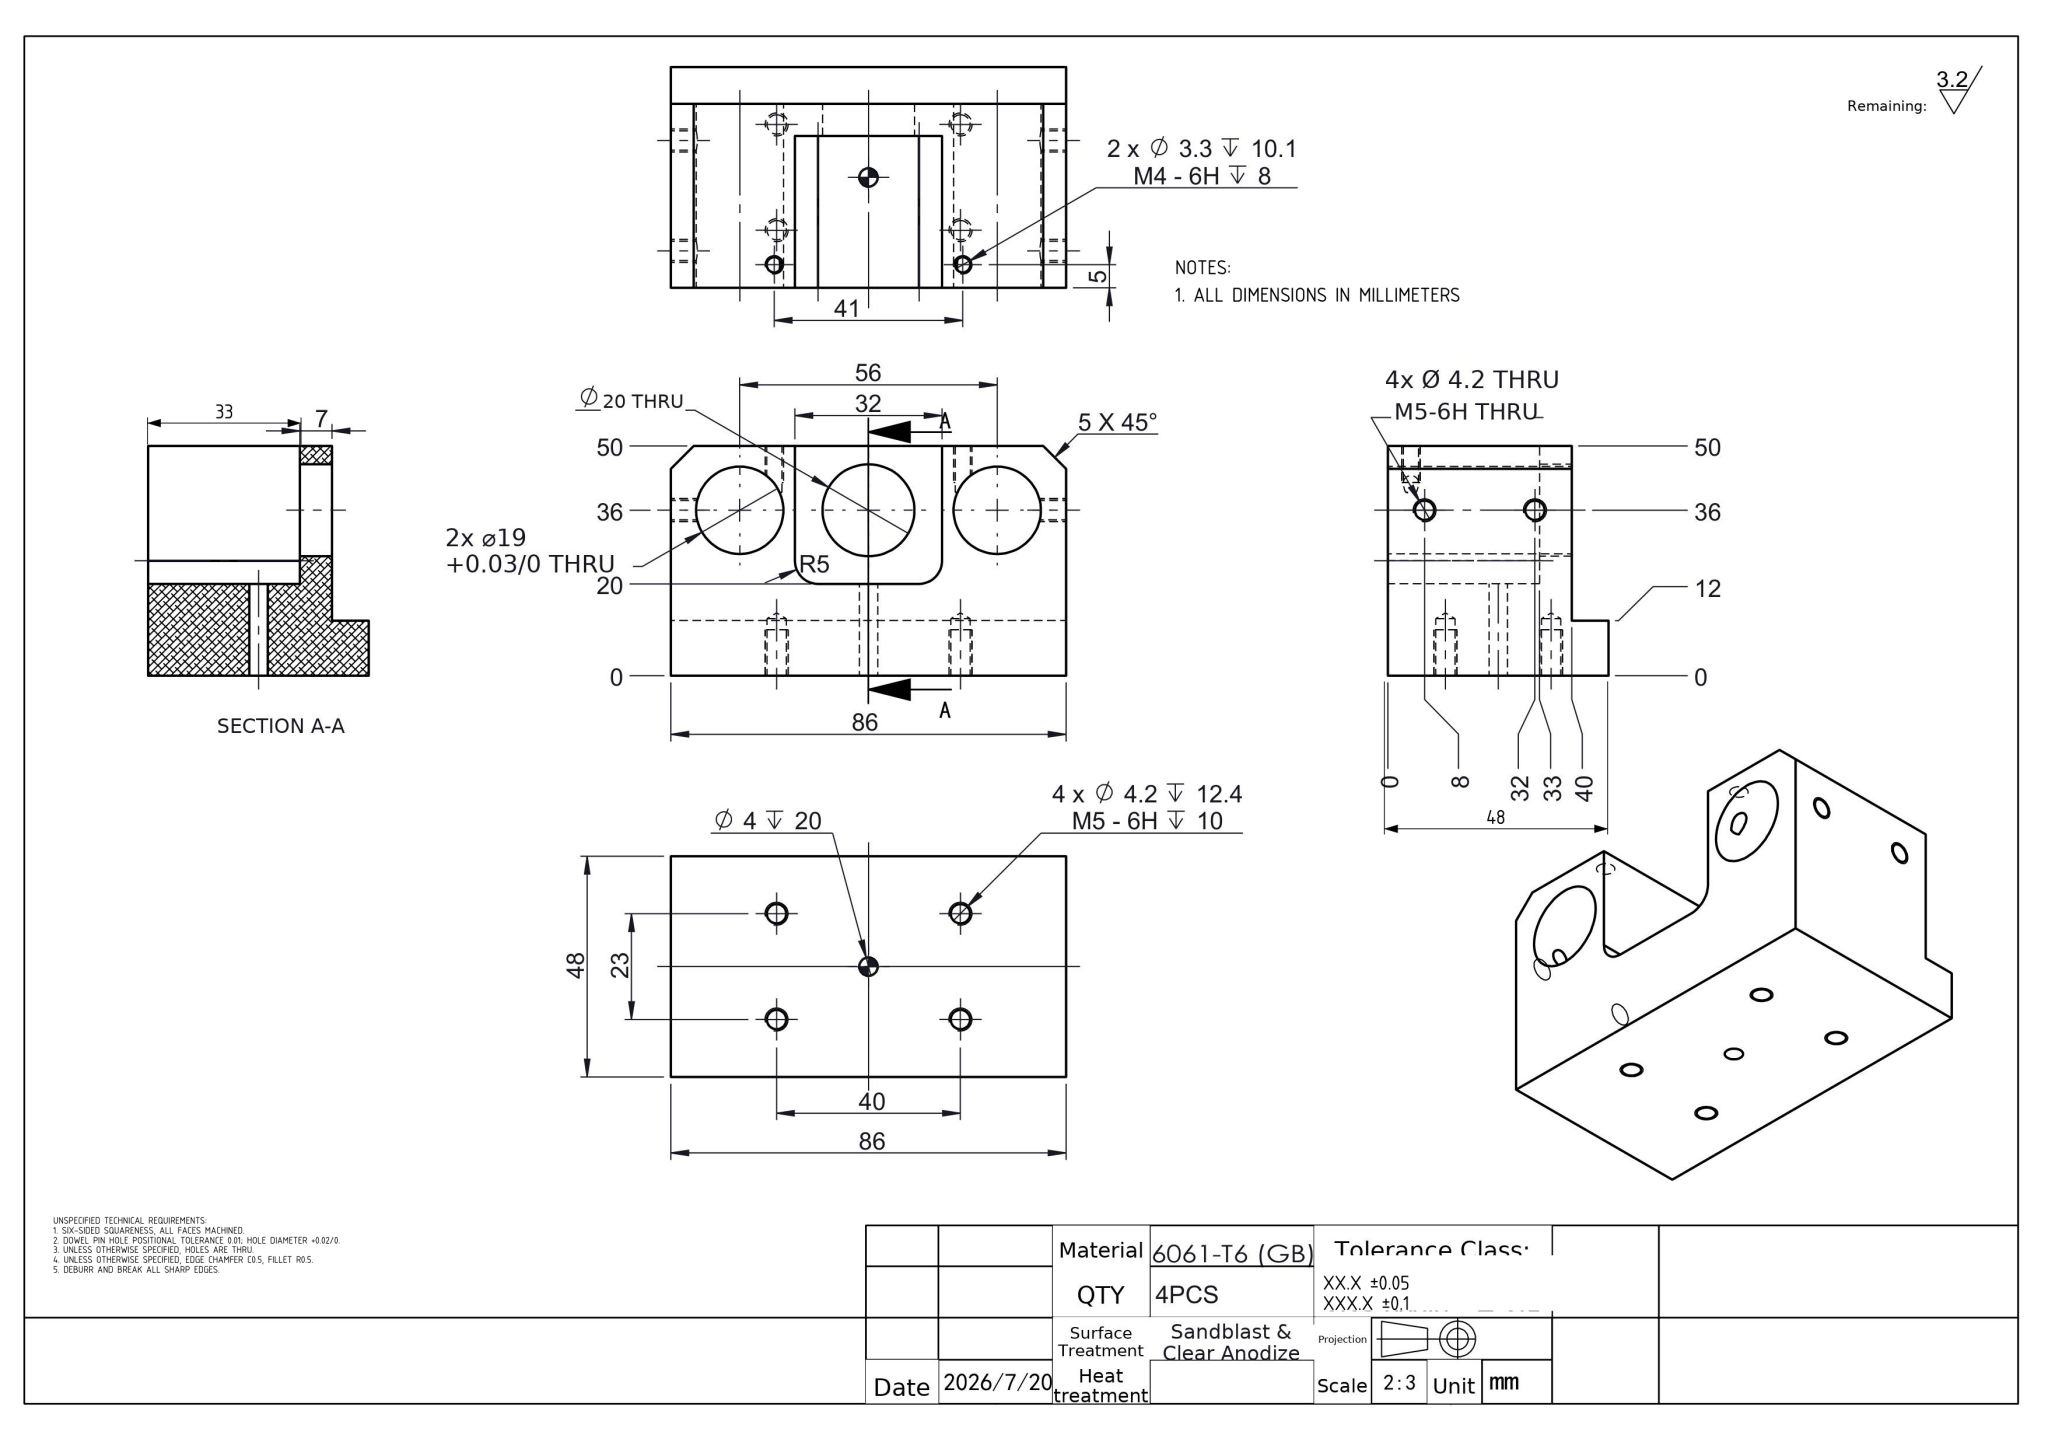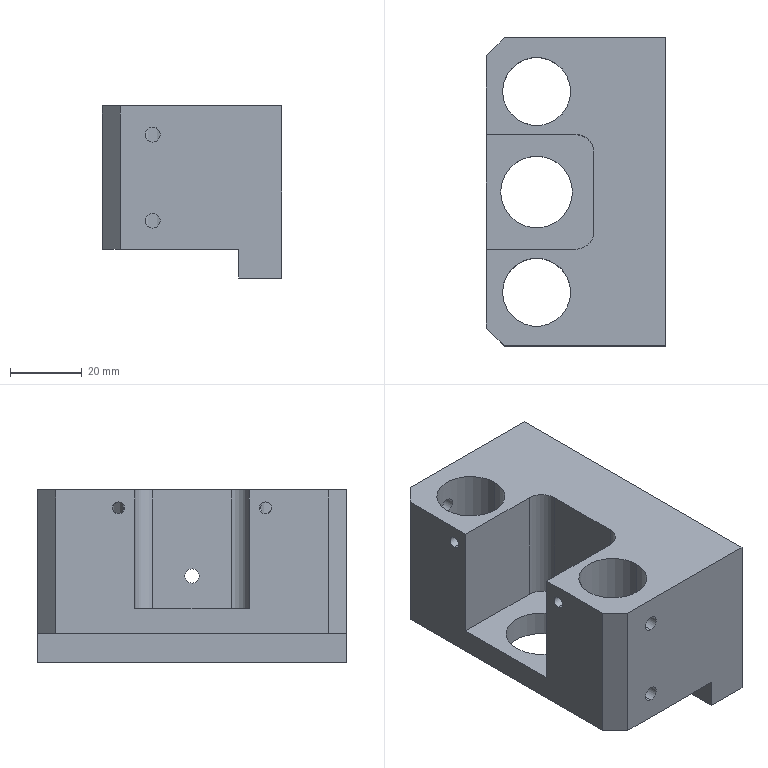Part | NX | mm | 1 solid | 54 faces | box 50 x 86 x 48 mm | volume 121637 mm3 | cylinder 30 | plane 14 | cone 10 | commonest cylinder face diameters 4.2 x16 3.3 x4 19 x4 4 x2 20 x2 10 x2